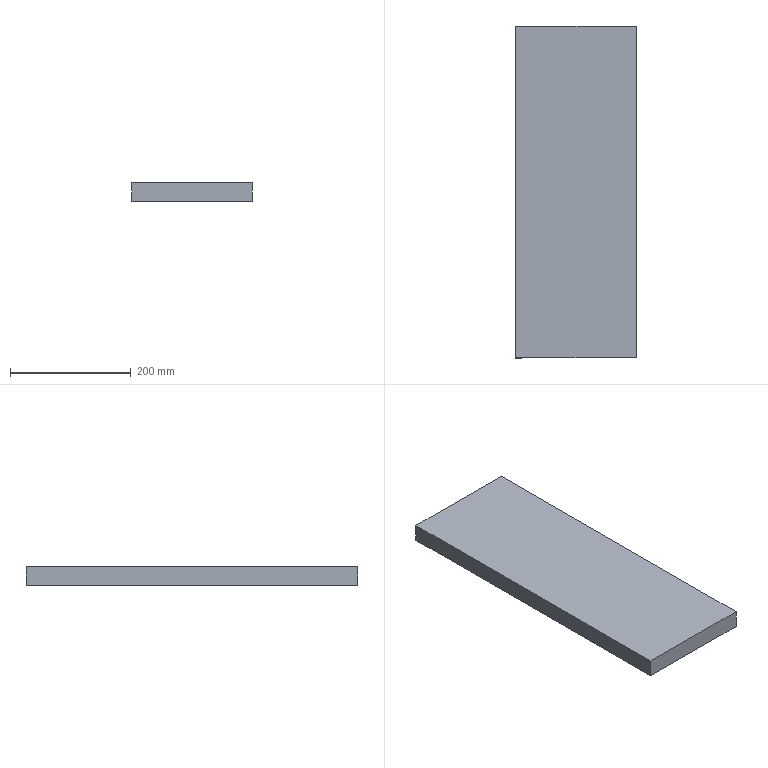Component | SolidWorks | BearingHousing-1_BearingHousingBasePlate-1 | 1 solid | 6 faces | box 200 x 550 x 30 mm | volume 3300000 mm3 | plane 6 | material Plain Carbon Steel
STEP:
#1=COLOUR_RGB('',0.7922,0.8196,0.9333);
#2=FILL_AREA_STYLE_COLOUR('',#1);
#3=FILL_AREA_STYLE('',(#2));
#4=SURFACE_STYLE_FILL_AREA(#3);
#5=SURFACE_SIDE_STYLE('',(#4));
#6=SURFACE_STYLE_USAGE(.BOTH.,#5);
#7=PRESENTATION_STYLE_ASSIGNMENT((#6));
#8=CARTESIAN_POINT('',(419.47,116.604,265.12));
#9=VERTEX_POINT('',#8);
#10=CARTESIAN_POINT('',(427.344,116.604,265.12));
#11=VERTEX_POINT('',#10);
#12=CARTESIAN_POINT('',(419.47,116.604,265.12));
#13=DIRECTION('',(1.,0.,-0.));
#14=VECTOR('',#13,39.37);
#15=LINE('',#12,#14);
#16=EDGE_CURVE('',#9,#11,#15,.T.);
#17=ORIENTED_EDGE('',*,*,#16,.F.);
#18=CARTESIAN_POINT('',(419.47,116.604,263.939));
#19=VERTEX_POINT('',#18);
#20=CARTESIAN_POINT('',(419.47,116.604,263.939));
#21=DIRECTION('',(0.,0.,1.));
#22=VECTOR('',#21,39.37);
#23=LINE('',#20,#22);
#24=EDGE_CURVE('',#19,#9,#23,.T.);
#25=ORIENTED_EDGE('',*,*,#24,.F.);
#26=CARTESIAN_POINT('',(427.344,116.604,263.939));
#27=VERTEX_POINT('',#26);
#28=CARTESIAN_POINT('',(419.47,116.604,263.939));
#29=DIRECTION('',(1.,0.,-0.));
#30=VECTOR('',#29,39.37);
#31=LINE('',#28,#30);
#32=EDGE_CURVE('',#19,#27,#31,.T.);
#33=ORIENTED_EDGE('',*,*,#32,.T.);
#34=CARTESIAN_POINT('',(427.344,116.604,263.939));
#35=DIRECTION('',(0.,0.,1.));
#36=VECTOR('',#35,39.37);
#37=LINE('',#34,#36);
#38=EDGE_CURVE('',#27,#11,#37,.T.);
#39=ORIENTED_EDGE('',*,*,#38,.T.);
#40=EDGE_LOOP('',(#17,#25,#33,#39));
#41=FACE_OUTER_BOUND('',#40,.T.);
#42=CARTESIAN_POINT('',(419.47,116.604,263.939));
#43=DIRECTION('',(0.,-1.,-0.));
#44=DIRECTION('',(1.,0.,-0.));
#45=AXIS2_PLACEMENT_3D('',#42,#43,#44);
#46=PLANE('',#45);
#47=ADVANCED_FACE('',(#41),#46,.T.);
#48=CARTESIAN_POINT('',(419.47,138.257,265.12));
#49=VERTEX_POINT('',#48);
#50=CARTESIAN_POINT('',(419.47,116.604,265.12));
#51=DIRECTION('',(0.,-1.,0.));
#52=VECTOR('',#51,39.37);
#53=LINE('',#50,#52);
#54=EDGE_CURVE('',#49,#9,#53,.T.);
#55=ORIENTED_EDGE('',*,*,#54,.F.);
#56=CARTESIAN_POINT('',(419.47,138.257,263.939));
#57=VERTEX_POINT('',#56);
#58=CARTESIAN_POINT('',(419.47,138.257,263.939));
#59=DIRECTION('',(0.,0.,1.));
#60=VECTOR('',#59,39.37);
#61=LINE('',#58,#60);
#62=EDGE_CURVE('',#57,#49,#61,.T.);
#63=ORIENTED_EDGE('',*,*,#62,.F.);
#64=CARTESIAN_POINT('',(419.47,116.604,263.939));
#65=DIRECTION('',(0.,-1.,0.));
#66=VECTOR('',#65,39.37);
#67=LINE('',#64,#66);
#68=EDGE_CURVE('',#57,#19,#67,.T.);
#69=ORIENTED_EDGE('',*,*,#68,.T.);
#70=ORIENTED_EDGE('',*,*,#24,.T.);
#71=EDGE_LOOP('',(#55,#63,#69,#70));
#72=FACE_OUTER_BOUND('',#71,.T.);
#73=CARTESIAN_POINT('',(419.47,116.604,263.939));
#74=DIRECTION('',(-1.,-0.,0.));
#75=DIRECTION('',(0.,-1.,0.));
#76=AXIS2_PLACEMENT_3D('',#73,#74,#75);
#77=PLANE('',#76);
#78=ADVANCED_FACE('',(#72),#77,.T.);
#79=CARTESIAN_POINT('',(427.344,138.257,265.12));
#80=VERTEX_POINT('',#79);
#81=CARTESIAN_POINT('',(419.47,138.257,265.12));
#82=DIRECTION('',(-1.,-0.,0.));
#83=VECTOR('',#82,39.37);
#84=LINE('',#81,#83);
#85=EDGE_CURVE('',#80,#49,#84,.T.);
#86=ORIENTED_EDGE('',*,*,#85,.F.);
#87=CARTESIAN_POINT('',(427.344,138.257,263.939));
#88=VERTEX_POINT('',#87);
#89=CARTESIAN_POINT('',(427.344,138.257,263.939));
#90=DIRECTION('',(0.,0.,1.));
#91=VECTOR('',#90,39.37);
#92=LINE('',#89,#91);
#93=EDGE_CURVE('',#88,#80,#92,.T.);
#94=ORIENTED_EDGE('',*,*,#93,.F.);
#95=CARTESIAN_POINT('',(419.47,138.257,263.939));
#96=DIRECTION('',(-1.,-0.,0.));
#97=VECTOR('',#96,39.37);
#98=LINE('',#95,#97);
#99=EDGE_CURVE('',#88,#57,#98,.T.);
#100=ORIENTED_EDGE('',*,*,#99,.T.);
#101=ORIENTED_EDGE('',*,*,#62,.T.);
#102=EDGE_LOOP('',(#86,#94,#100,#101));
#103=FACE_OUTER_BOUND('',#102,.T.);
#104=CARTESIAN_POINT('',(419.47,138.257,263.939));
#105=DIRECTION('',(-0.,1.,-0.));
#106=DIRECTION('',(-1.,-0.,0.));
#107=AXIS2_PLACEMENT_3D('',#104,#105,#106);
#108=PLANE('',#107);
#109=ADVANCED_FACE('',(#103),#108,.T.);
#110=CARTESIAN_POINT('',(427.344,116.604,265.12));
#111=DIRECTION('',(-0.,1.,0.));
#112=VECTOR('',#111,39.37);
#113=LINE('',#110,#112);
#114=EDGE_CURVE('',#11,#80,#113,.T.);
#115=ORIENTED_EDGE('',*,*,#114,.F.);
#116=ORIENTED_EDGE('',*,*,#38,.F.);
#117=CARTESIAN_POINT('',(427.344,116.604,263.939));
#118=DIRECTION('',(-0.,1.,0.));
#119=VECTOR('',#118,39.37);
#120=LINE('',#117,#119);
#121=EDGE_CURVE('',#27,#88,#120,.T.);
#122=ORIENTED_EDGE('',*,*,#121,.T.);
#123=ORIENTED_EDGE('',*,*,#93,.T.);
#124=EDGE_LOOP('',(#115,#116,#122,#123));
#125=FACE_OUTER_BOUND('',#124,.T.);
#126=CARTESIAN_POINT('',(427.344,116.604,263.939));
#127=DIRECTION('',(1.,0.,-0.));
#128=DIRECTION('',(-0.,1.,0.));
#129=AXIS2_PLACEMENT_3D('',#126,#127,#128);
#130=PLANE('',#129);
#131=ADVANCED_FACE('',(#125),#130,.T.);
#132=ORIENTED_EDGE('',*,*,#32,.F.);
#133=ORIENTED_EDGE('',*,*,#68,.F.);
#134=ORIENTED_EDGE('',*,*,#99,.F.);
#135=ORIENTED_EDGE('',*,*,#121,.F.);
#136=EDGE_LOOP('',(#132,#133,#134,#135));
#137=FACE_OUTER_BOUND('',#136,.T.);
#138=CARTESIAN_POINT('',(419.47,116.604,263.939));
#139=DIRECTION('',(0.,0.,1.));
#140=DIRECTION('',(1.,0.,-0.));
#141=AXIS2_PLACEMENT_3D('',#138,#139,#140);
#142=PLANE('',#141);
#143=ADVANCED_FACE('',(#137),#142,.F.);
#144=ORIENTED_EDGE('',*,*,#16,.T.);
#145=ORIENTED_EDGE('',*,*,#114,.T.);
#146=ORIENTED_EDGE('',*,*,#85,.T.);
#147=ORIENTED_EDGE('',*,*,#54,.T.);
#148=EDGE_LOOP('',(#144,#145,#146,#147));
#149=FACE_OUTER_BOUND('',#148,.T.);
#150=CARTESIAN_POINT('',(419.47,116.604,265.12));
#151=DIRECTION('',(0.,0.,1.));
#152=DIRECTION('',(1.,0.,-0.));
#153=AXIS2_PLACEMENT_3D('',#150,#151,#152);
#154=PLANE('',#153);
#155=ADVANCED_FACE('',(#149),#154,.T.);
#156=CLOSED_SHELL('',(#47,#78,#109,#131,#143,#155));
#157=MANIFOLD_SOLID_BREP('',#156);
#158=STYLED_ITEM('',(#7),#157);
#159=PRESENTATION_LAYER_ASSIGNMENT('','',(#158));
#160=CARTESIAN_POINT('',(0.,0.,0.));
#161=DIRECTION('',(0.,0.,1.));
#162=DIRECTION('',(1.,0.,0.));
#163=AXIS2_PLACEMENT_3D('',#160,#161,#162);
#164=(LENGTH_UNIT()NAMED_UNIT(*)SI_UNIT($,.METRE.));
#165=LENGTH_MEASURE_WITH_UNIT(LENGTH_MEASURE(0.0254),#164);
#166=DIMENSIONAL_EXPONENTS(1.,0.,0.,0.,0.,0.,0.);
#167=(CONVERSION_BASED_UNIT('',#165)LENGTH_UNIT()NAMED_UNIT(#166));
#168=UNCERTAINTY_MEASURE_WITH_UNIT(LENGTH_MEASURE(0.00001),#167,'','');
#169=(NAMED_UNIT(*)PLANE_ANGLE_UNIT()SI_UNIT($,.RADIAN.));
#170=(NAMED_UNIT(*)SI_UNIT($,.STERADIAN.)SOLID_ANGLE_UNIT());
#171=(GEOMETRIC_REPRESENTATION_CONTEXT(3)GLOBAL_UNCERTAINTY_ASSIGNED_CONTEXT((#168))GLOBAL_UNIT_ASSIGNED_CONTEXT((#167,#169,#170))REPRESENTATION_CONTEXT('',''));
#172=ADVANCED_BREP_SHAPE_REPRESENTATION('',(#157,#163),#171);
#173=(LENGTH_UNIT()NAMED_UNIT(*)SI_UNIT($,.METRE.));
#174=LENGTH_MEASURE_WITH_UNIT(LENGTH_MEASURE(0.0254),#173);
#175=DIMENSIONAL_EXPONENTS(1.,0.,0.,0.,0.,0.,0.);
#176=(CONVERSION_BASED_UNIT('',#174)LENGTH_UNIT()NAMED_UNIT(#175));
#177=UNCERTAINTY_MEASURE_WITH_UNIT(LENGTH_MEASURE(0.00001),#176,'','');
#178=(NAMED_UNIT(*)PLANE_ANGLE_UNIT()SI_UNIT($,.RADIAN.));
#179=(NAMED_UNIT(*)SI_UNIT($,.STERADIAN.)SOLID_ANGLE_UNIT());
#180=(GEOMETRIC_REPRESENTATION_CONTEXT(3)GLOBAL_UNCERTAINTY_ASSIGNED_CONTEXT((#177))GLOBAL_UNIT_ASSIGNED_CONTEXT((#176,#178,#179))REPRESENTATION_CONTEXT('',''));
#181=MECHANICAL_DESIGN_GEOMETRIC_PRESENTATION_REPRESENTATION('',(#158),#180);